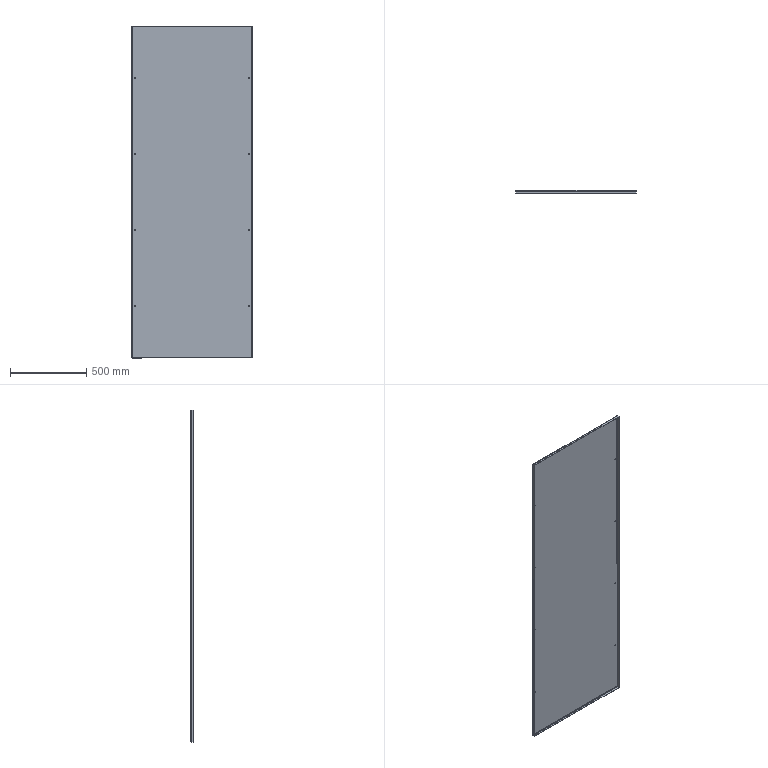Component | SolidWorks | SidePlate(Item17)-1 | 1 solid | 54 faces | volume 3612966 mm3 | cylinder 24 | plane 22 | spline 8 | commonest cylinder face diameters 6.5 x16 10 x4 6 x4 | material Plain Carbon Steel